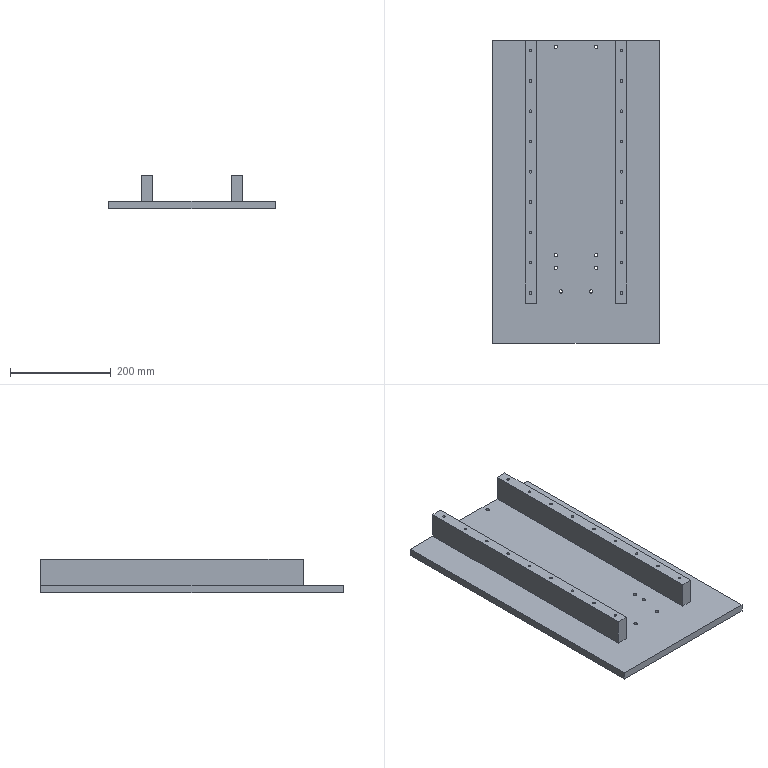Component | NX | GUIDE_RAIL_BASE | 1 solid | 58 faces | volume 4149394 mm3 | plane 32 | cylinder 26 | commonest cylinder face diameters 5 x18 6.8 x8